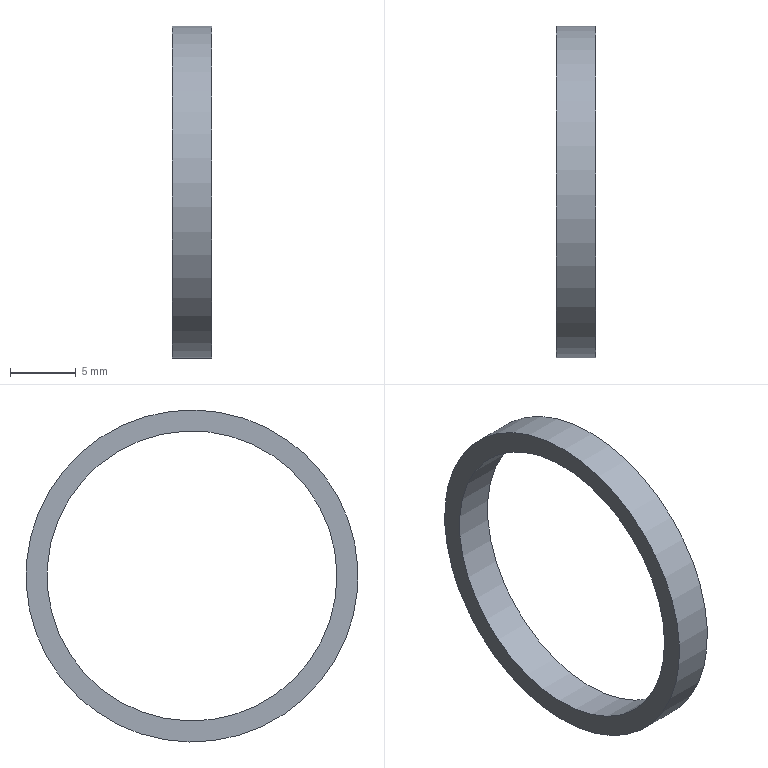Component | NX | PISTON_RING | 1 solid | 4 faces | volume 356 mm3 | cylinder 2 | plane 2 | commonest cylinder face diameters 25.2 x1 22 x1